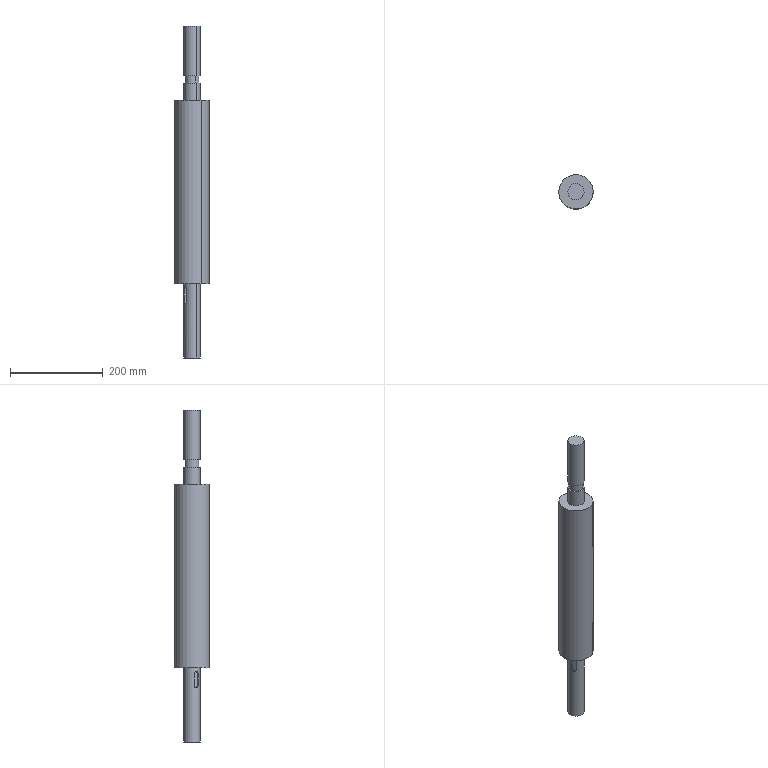Component | SolidWorks | AirShaft-1 | 1 solid | 27 faces | box 74 x 74 x 715 mm | volume 1997791 mm3 | cylinder 14 | plane 9 | cone 4 | commonest cylinder face diameters 35 x6 10.2 x2 30 x2 74 x2 10 x2
build123d program:
from build123d import *

# Parameters (mm, degrees)
SKETCH2_R                              = 17.5
BOSS_EXTRUDE1_DEPTH                    = 160
CUT_EXTRUDE1_REACH                     = 364.802
CUT_EXTRUDE1_END_RADIUS                = 17.5
F_10_2_10_2_DIAMETER_HOLE1_D           = 10.2
F_10_2_10_2_DIAMETER_HOLE1_DEPTH       = 38.75
F_10_2_10_2_DIAMETER_HOLE1_CSINK_D     = 12.05
F_10_2_10_2_DIAMETER_HOLE1_CSINK_ANGLE = 90
F_10_2_10_2_DIAMETER_HOLE1_TIP         = 3.064


with BuildPart() as part:
    # Sketch1 → Revolve1 (revolve)
    with BuildSketch(Plane(origin=(0, 0, 0), x_dir=(-1, 0, 0), z_dir=(0, 0, -1)), mode=Mode.PRIVATE) as revolve1_sk:
        Polygon((-357.5, 17.5), (-357.5, 0), (197.5, 0), (197.5, 37), (-197.5, 37), (-197.5, 17.5), (-234.5, 17.5), (-234.5, 15), (-250.5, 15), (-250.5, 17.5), align=None)
    revolve(revolve1_sk.sketch.rotate(Axis((357.5, 0, 0), (-1, 0, 0)), 270), axis=Axis((357.5, 0, 0), (-1, 0, 0)))

    # Sketch2 → Boss-Extrude1 (add)
    with BuildSketch(Plane.ZY.offset(197.5)):
        Circle(SKETCH2_R)
    extrude(amount=BOSS_EXTRUDE1_DEPTH)

    # Cut-Extrude1: up to this cylinder (the profile starts inside it)
    cut_extrude1_end = Plane(origin=(-223, 0, 0), z_dir=(1, 0, 0)) * Cylinder(CUT_EXTRUDE1_END_RADIUS, 765.604, mode=Mode.PRIVATE)
    # Sketch3 → Cut-Extrude1 (cut, up to the surface)
    with BuildSketch(Plane.XZ.offset(-12.5), mode=Mode.PRIVATE) as cut_extrude1_sk1:
        with BuildLine():
            Line((-235.5, -5), (-210.5, -5))
            ThreePointArc((-210.5, -5), (-205.5, 0), (-210.5, 5))
            Line((-210.5, 5), (-235.5, 5))
            ThreePointArc((-235.5, 5), (-240.5, 0), (-235.5, -5))
        make_face()
    cut_extrude1_tool1 = extrude(cut_extrude1_sk1.sketch, amount=-CUT_EXTRUDE1_REACH, mode=Mode.PRIVATE) & cut_extrude1_end
    add(cut_extrude1_tool1.solids().sort_by_distance((-223, 12.5, 0))[0], mode=Mode.SUBTRACT)

    # 10.2 _10.2_ Diameter Hole1
    with Locations(Plane.ZY.offset(357.5)):
        with Locations((0, 0)):
            CounterSinkHole(F_10_2_10_2_DIAMETER_HOLE1_D / 2, F_10_2_10_2_DIAMETER_HOLE1_CSINK_D / 2, depth=F_10_2_10_2_DIAMETER_HOLE1_DEPTH, counter_sink_angle=F_10_2_10_2_DIAMETER_HOLE1_CSINK_ANGLE)
            with Locations((0, 0, -(F_10_2_10_2_DIAMETER_HOLE1_DEPTH + F_10_2_10_2_DIAMETER_HOLE1_TIP / 2))):  # 118° drill point
                Cone(0, F_10_2_10_2_DIAMETER_HOLE1_D / 2, F_10_2_10_2_DIAMETER_HOLE1_TIP, mode=Mode.SUBTRACT)


solid = part.part

# Placed as in the assembly
solid = solid.moved(Location((-345, -229, 12.5), (90, 31.701, 90)))
STEP:
#1=COLOUR_RGB('',0.7922,0.8196,0.9333);
#2=FILL_AREA_STYLE_COLOUR('',#1);
#3=FILL_AREA_STYLE('',(#2));
#4=SURFACE_STYLE_FILL_AREA(#3);
#5=SURFACE_SIDE_STYLE('',(#4));
#6=SURFACE_STYLE_USAGE(.BOTH.,#5);
#7=PRESENTATION_STYLE_ASSIGNMENT((#6));
#8=CARTESIAN_POINT('',(-13.688,-8.845,-13.546));
#9=VERTEX_POINT('',#8);
#10=CARTESIAN_POINT('',(-13.477,-9.187,-13.546));
#11=VERTEX_POINT('',#10);
#12=CARTESIAN_POINT('',(-13.583,-9.016,-13.546));
#13=DIRECTION('',(0.,0.,-1.));
#14=DIRECTION('',(0.5255,-0.8508,0.));
#15=AXIS2_PLACEMENT_3D('',#12,#13,#14);
#16=CIRCLE('',#15,0.2008);
#17=EDGE_CURVE('',#9,#11,#16,.T.);
#18=ORIENTED_EDGE('',*,*,#17,.F.);
#19=CARTESIAN_POINT('',(-13.707,-8.814,-13.583));
#20=VERTEX_POINT('',#19);
#21=CARTESIAN_POINT('',(-13.707,-8.814,-13.583));
#22=DIRECTION('',(-0.3716,0.6016,-0.7071));
#23=VECTOR('',#22,39.37);
#24=LINE('',#21,#23);
#25=EDGE_CURVE('',#9,#20,#24,.T.);
#26=ORIENTED_EDGE('',*,*,#25,.T.);
#27=CARTESIAN_POINT('',(-13.458,-9.218,-13.583));
#28=VERTEX_POINT('',#27);
#29=CARTESIAN_POINT('',(-13.583,-9.016,-13.583));
#30=DIRECTION('',(0.,0.,-1.));
#31=DIRECTION('',(0.5255,-0.8508,0.));
#32=AXIS2_PLACEMENT_3D('',#29,#30,#31);
#33=CIRCLE('',#32,0.2372);
#34=EDGE_CURVE('',#20,#28,#33,.T.);
#35=ORIENTED_EDGE('',*,*,#34,.T.);
#36=CARTESIAN_POINT('',(-13.458,-9.218,-13.583));
#37=DIRECTION('',(0.3716,-0.6016,-0.7071));
#38=VECTOR('',#37,39.37);
#39=LINE('',#36,#38);
#40=EDGE_CURVE('',#11,#28,#39,.T.);
#41=ORIENTED_EDGE('',*,*,#40,.F.);
#42=EDGE_LOOP('',(#18,#26,#35,#41));
#43=FACE_OUTER_BOUND('',#42,.T.);
#44=CARTESIAN_POINT('',(-13.583,-9.016,-13.583));
#45=DIRECTION('',(0.,0.,-1.));
#46=DIRECTION('',(0.5255,-0.8508,0.));
#47=AXIS2_PLACEMENT_3D('',#44,#45,#46);
#48=CONICAL_SURFACE('',#47,0.2372,0.7854);
#49=ADVANCED_FACE('',(#43),#48,.F.);
#50=CARTESIAN_POINT('',(-13.688,-8.845,-12.057));
#51=VERTEX_POINT('',#50);
#52=CARTESIAN_POINT('',(-13.477,-9.187,-12.057));
#53=VERTEX_POINT('',#52);
#54=CARTESIAN_POINT('',(-13.583,-9.016,-12.057));
#55=DIRECTION('',(0.,0.,-1.));
#56=DIRECTION('',(0.5255,-0.8508,0.));
#57=AXIS2_PLACEMENT_3D('',#54,#55,#56);
#58=CIRCLE('',#57,0.2008);
#59=EDGE_CURVE('',#51,#53,#58,.T.);
#60=ORIENTED_EDGE('',*,*,#59,.F.);
#61=CARTESIAN_POINT('',(-13.688,-8.845,-13.583));
#62=DIRECTION('',(0.,0.,-1.));
#63=VECTOR('',#62,39.37);
#64=LINE('',#61,#63);
#65=EDGE_CURVE('',#51,#9,#64,.T.);
#66=ORIENTED_EDGE('',*,*,#65,.T.);
#67=ORIENTED_EDGE('',*,*,#17,.T.);
#68=CARTESIAN_POINT('',(-13.477,-9.187,-13.583));
#69=DIRECTION('',(0.,0.,-1.));
#70=VECTOR('',#69,39.37);
#71=LINE('',#68,#70);
#72=EDGE_CURVE('',#53,#11,#71,.T.);
#73=ORIENTED_EDGE('',*,*,#72,.F.);
#74=EDGE_LOOP('',(#60,#66,#67,#73));
#75=FACE_OUTER_BOUND('',#74,.T.);
#76=CARTESIAN_POINT('',(-13.583,-9.016,-13.583));
#77=DIRECTION('',(0.,0.,-1.));
#78=DIRECTION('',(0.5255,-0.8508,0.));
#79=AXIS2_PLACEMENT_3D('',#76,#77,#78);
#80=CYLINDRICAL_SURFACE('',#79,0.2008);
#81=ADVANCED_FACE('',(#75),#80,.F.);
#82=CARTESIAN_POINT('',(-13.583,-9.016,-11.936));
#83=VERTEX_POINT('',#82);
#84=CARTESIAN_POINT('',(-13.477,-9.187,-12.057));
#85=DIRECTION('',(0.4504,-0.7293,-0.515));
#86=VECTOR('',#85,39.37);
#87=LINE('',#84,#86);
#88=EDGE_CURVE('',#83,#53,#87,.T.);
#89=ORIENTED_EDGE('',*,*,#88,.F.);
#90=CARTESIAN_POINT('',(-13.688,-8.845,-12.057));
#91=DIRECTION('',(-0.4504,0.7293,-0.515));
#92=VECTOR('',#91,39.37);
#93=LINE('',#90,#92);
#94=EDGE_CURVE('',#83,#51,#93,.T.);
#95=ORIENTED_EDGE('',*,*,#94,.T.);
#96=ORIENTED_EDGE('',*,*,#59,.T.);
#97=EDGE_LOOP('',(#89,#95,#96));
#98=FACE_OUTER_BOUND('',#97,.T.);
#99=CARTESIAN_POINT('',(-13.583,-9.016,-12.057));
#100=DIRECTION('',(0.,0.,-1.));
#101=DIRECTION('',(0.5255,-0.8508,0.));
#102=AXIS2_PLACEMENT_3D('',#99,#100,#101);
#103=CONICAL_SURFACE('',#102,0.2008,1.03);
#104=ADVANCED_FACE('',(#98),#103,.F.);
#105=CARTESIAN_POINT('',(-14.041,-9.53,-7.795));
#106=VERTEX_POINT('',#105);
#107=CARTESIAN_POINT('',(-14.041,-9.53,-8.78));
#108=VERTEX_POINT('',#107);
#109=CARTESIAN_POINT('',(-14.041,-9.53,-13.583));
#110=DIRECTION('',(0.,0.,-1.));
#111=VECTOR('',#110,39.37);
#112=LINE('',#109,#111);
#113=EDGE_CURVE('',#106,#108,#112,.T.);
#114=ORIENTED_EDGE('',*,*,#113,.T.);
#115=CARTESIAN_POINT('',(-14.248,-9.195,-8.78));
#116=VERTEX_POINT('',#115);
#117=CARTESIAN_POINT('',(-14.041,-9.53,-8.78));
#118=CARTESIAN_POINT('',(-14.041,-9.53,-8.793));
#119=CARTESIAN_POINT('',(-14.042,-9.529,-8.805));
#120=CARTESIAN_POINT('',(-14.046,-9.526,-8.831));
#121=CARTESIAN_POINT('',(-14.049,-9.523,-8.843));
#122=CARTESIAN_POINT('',(-14.056,-9.516,-8.867));
#123=CARTESIAN_POINT('',(-14.061,-9.512,-8.878));
#124=CARTESIAN_POINT('',(-14.071,-9.501,-8.9));
#125=CARTESIAN_POINT('',(-14.077,-9.495,-8.91));
#126=CARTESIAN_POINT('',(-14.09,-9.482,-8.928));
#127=CARTESIAN_POINT('',(-14.097,-9.475,-8.936));
#128=CARTESIAN_POINT('',(-14.111,-9.458,-8.95));
#129=CARTESIAN_POINT('',(-14.118,-9.449,-8.956));
#130=CARTESIAN_POINT('',(-14.129,-9.435,-8.964));
#131=CARTESIAN_POINT('',(-14.133,-9.43,-8.966));
#132=CARTESIAN_POINT('',(-14.14,-9.42,-8.97));
#133=CARTESIAN_POINT('',(-14.144,-9.415,-8.971));
#134=CARTESIAN_POINT('',(-14.155,-9.4,-8.975));
#135=CARTESIAN_POINT('',(-14.162,-9.389,-8.976));
#136=CARTESIAN_POINT('',(-14.176,-9.367,-8.976));
#137=CARTESIAN_POINT('',(-14.182,-9.356,-8.975));
#138=CARTESIAN_POINT('',(-14.194,-9.333,-8.97));
#139=CARTESIAN_POINT('',(-14.2,-9.322,-8.966));
#140=CARTESIAN_POINT('',(-14.21,-9.301,-8.956));
#141=CARTESIAN_POINT('',(-14.215,-9.29,-8.95));
#142=CARTESIAN_POINT('',(-14.223,-9.27,-8.936));
#143=CARTESIAN_POINT('',(-14.227,-9.261,-8.928));
#144=CARTESIAN_POINT('',(-14.233,-9.243,-8.91));
#145=CARTESIAN_POINT('',(-14.236,-9.235,-8.9));
#146=CARTESIAN_POINT('',(-14.24,-9.221,-8.879));
#147=CARTESIAN_POINT('',(-14.242,-9.215,-8.867));
#148=CARTESIAN_POINT('',(-14.245,-9.205,-8.843));
#149=CARTESIAN_POINT('',(-14.246,-9.202,-8.831));
#150=CARTESIAN_POINT('',(-14.248,-9.197,-8.806));
#151=CARTESIAN_POINT('',(-14.248,-9.195,-8.793));
#152=CARTESIAN_POINT('',(-14.248,-9.195,-8.78));
#153=B_SPLINE_CURVE_WITH_KNOTS('',3,(#117,#118,#119,#120,#121,#122,#123,#124,#125,#126,#127,#128,#129,#130,#131,#132,#133,#134,#135,#136,#137,#138,#139,#140,#141,#142,#143,#144,#145,#146,#147,#148,#149,#150,#151,#152),.UNSPECIFIED.,.F.,.F.,(4,2,2,2,2,2,2,2,2,2,2,2,2,2,2,2,2,4),(0.,0.0009818,0.001964,0.002945,0.003927,0.004909,0.005891,0.006382,0.006873,0.007855,0.008836,0.009818,0.0108,0.01178,0.01276,0.01375,0.01473,0.01571),.UNSPECIFIED.);
#154=EDGE_CURVE('',#108,#116,#153,.T.);
#155=ORIENTED_EDGE('',*,*,#154,.T.);
#156=CARTESIAN_POINT('',(-14.248,-9.195,-7.795));
#157=VERTEX_POINT('',#156);
#158=CARTESIAN_POINT('',(-14.248,-9.195,-13.583));
#159=DIRECTION('',(-0.,-0.,1.));
#160=VECTOR('',#159,39.37);
#161=LINE('',#158,#160);
#162=EDGE_CURVE('',#116,#157,#161,.T.);
#163=ORIENTED_EDGE('',*,*,#162,.T.);
#164=CARTESIAN_POINT('',(-14.248,-9.195,-7.795));
#165=CARTESIAN_POINT('',(-14.248,-9.195,-7.782));
#166=CARTESIAN_POINT('',(-14.248,-9.197,-7.769));
#167=CARTESIAN_POINT('',(-14.246,-9.202,-7.744));
#168=CARTESIAN_POINT('',(-14.245,-9.205,-7.732));
#169=CARTESIAN_POINT('',(-14.242,-9.215,-7.708));
#170=CARTESIAN_POINT('',(-14.24,-9.221,-7.697));
#171=CARTESIAN_POINT('',(-14.236,-9.235,-7.675));
#172=CARTESIAN_POINT('',(-14.233,-9.243,-7.665));
#173=CARTESIAN_POINT('',(-14.227,-9.261,-7.647));
#174=CARTESIAN_POINT('',(-14.223,-9.27,-7.639));
#175=CARTESIAN_POINT('',(-14.215,-9.29,-7.625));
#176=CARTESIAN_POINT('',(-14.21,-9.3,-7.618));
#177=CARTESIAN_POINT('',(-14.203,-9.317,-7.611));
#178=CARTESIAN_POINT('',(-14.2,-9.322,-7.609));
#179=CARTESIAN_POINT('',(-14.194,-9.333,-7.605));
#180=CARTESIAN_POINT('',(-14.191,-9.339,-7.604));
#181=CARTESIAN_POINT('',(-14.182,-9.356,-7.6));
#182=CARTESIAN_POINT('',(-14.176,-9.367,-7.598));
#183=CARTESIAN_POINT('',(-14.162,-9.389,-7.598));
#184=CARTESIAN_POINT('',(-14.155,-9.4,-7.6));
#185=CARTESIAN_POINT('',(-14.14,-9.42,-7.605));
#186=CARTESIAN_POINT('',(-14.133,-9.43,-7.608));
#187=CARTESIAN_POINT('',(-14.118,-9.449,-7.618));
#188=CARTESIAN_POINT('',(-14.111,-9.458,-7.625));
#189=CARTESIAN_POINT('',(-14.097,-9.474,-7.639));
#190=CARTESIAN_POINT('',(-14.09,-9.482,-7.647));
#191=CARTESIAN_POINT('',(-14.077,-9.495,-7.665));
#192=CARTESIAN_POINT('',(-14.071,-9.501,-7.675));
#193=CARTESIAN_POINT('',(-14.061,-9.512,-7.696));
#194=CARTESIAN_POINT('',(-14.056,-9.516,-7.708));
#195=CARTESIAN_POINT('',(-14.049,-9.523,-7.731));
#196=CARTESIAN_POINT('',(-14.046,-9.526,-7.744));
#197=CARTESIAN_POINT('',(-14.042,-9.529,-7.769));
#198=CARTESIAN_POINT('',(-14.041,-9.53,-7.782));
#199=CARTESIAN_POINT('',(-14.041,-9.53,-7.795));
#200=B_SPLINE_CURVE_WITH_KNOTS('',3,(#164,#165,#166,#167,#168,#169,#170,#171,#172,#173,#174,#175,#176,#177,#178,#179,#180,#181,#182,#183,#184,#185,#186,#187,#188,#189,#190,#191,#192,#193,#194,#195,#196,#197,#198,#199),.UNSPECIFIED.,.F.,.F.,(4,2,2,2,2,2,2,2,2,2,2,2,2,2,2,2,2,4),(0.,0.0009818,0.001964,0.002945,0.003927,0.004909,0.005891,0.006382,0.006873,0.007855,0.008836,0.009818,0.0108,0.01178,0.01276,0.01375,0.01473,0.01571),.UNSPECIFIED.);
#201=EDGE_CURVE('',#157,#106,#200,.T.);
#202=ORIENTED_EDGE('',*,*,#201,.T.);
#203=EDGE_LOOP('',(#114,#155,#163,#202));
#204=FACE_BOUND('',#203,.T.);
#205=CARTESIAN_POINT('',(-13.221,-9.602,-13.583));
#206=VERTEX_POINT('',#205);
#207=CARTESIAN_POINT('',(-13.945,-8.43,-13.583));
#208=VERTEX_POINT('',#207);
#209=CARTESIAN_POINT('',(-13.583,-9.016,-13.583));
#210=DIRECTION('',(0.,0.,-1.));
#211=DIRECTION('',(0.5255,-0.8508,0.));
#212=AXIS2_PLACEMENT_3D('',#209,#210,#211);
#213=CIRCLE('',#212,0.689);
#214=EDGE_CURVE('',#206,#208,#213,.T.);
#215=ORIENTED_EDGE('',*,*,#214,.F.);
#216=CARTESIAN_POINT('',(-13.221,-9.602,-7.283));
#217=VERTEX_POINT('',#216);
#218=CARTESIAN_POINT('',(-13.221,-9.602,-13.583));
#219=DIRECTION('',(-0.,-0.,1.));
#220=VECTOR('',#219,39.37);
#221=LINE('',#218,#220);
#222=EDGE_CURVE('',#206,#217,#221,.T.);
#223=ORIENTED_EDGE('',*,*,#222,.T.);
#224=CARTESIAN_POINT('',(-13.945,-8.43,-7.283));
#225=VERTEX_POINT('',#224);
#226=CARTESIAN_POINT('',(-13.583,-9.016,-7.283));
#227=DIRECTION('',(0.,0.,-1.));
#228=DIRECTION('',(0.5255,-0.8508,0.));
#229=AXIS2_PLACEMENT_3D('',#226,#227,#228);
#230=CIRCLE('',#229,0.689);
#231=EDGE_CURVE('',#217,#225,#230,.T.);
#232=ORIENTED_EDGE('',*,*,#231,.T.);
#233=CARTESIAN_POINT('',(-13.945,-8.43,-13.583));
#234=DIRECTION('',(-0.,-0.,1.));
#235=VECTOR('',#234,39.37);
#236=LINE('',#233,#235);
#237=EDGE_CURVE('',#208,#225,#236,.T.);
#238=ORIENTED_EDGE('',*,*,#237,.F.);
#239=EDGE_LOOP('',(#215,#223,#232,#238));
#240=FACE_OUTER_BOUND('',#239,.T.);
#241=CARTESIAN_POINT('',(-13.583,-9.016,-13.583));
#242=DIRECTION('',(-0.,-0.,1.));
#243=DIRECTION('',(-0.5255,0.8508,0.));
#244=AXIS2_PLACEMENT_3D('',#241,#242,#243);
#245=CYLINDRICAL_SURFACE('',#244,0.689);
#246=ADVANCED_FACE('',(#204,#240),#245,.T.);
#247=CARTESIAN_POINT('',(-13.272,-9.518,10.354));
#248=VERTEX_POINT('',#247);
#249=CARTESIAN_POINT('',(-13.893,-8.513,10.354));
#250=VERTEX_POINT('',#249);
#251=CARTESIAN_POINT('',(-13.583,-9.016,10.354));
#252=DIRECTION('',(0.,0.,-1.));
#253=DIRECTION('',(0.5255,-0.8508,0.));
#254=AXIS2_PLACEMENT_3D('',#251,#252,#253);
#255=CIRCLE('',#254,0.5906);
#256=EDGE_CURVE('',#248,#250,#255,.T.);
#257=ORIENTED_EDGE('',*,*,#256,.T.);
#258=CARTESIAN_POINT('',(-13.893,-8.513,9.724));
#259=VERTEX_POINT('',#258);
#260=CARTESIAN_POINT('',(-13.893,-8.513,14.567));
#261=DIRECTION('',(0.,0.,-1.));
#262=VECTOR('',#261,39.37);
#263=LINE('',#260,#262);
#264=EDGE_CURVE('',#250,#259,#263,.T.);
#265=ORIENTED_EDGE('',*,*,#264,.T.);
#266=CARTESIAN_POINT('',(-13.272,-9.518,9.724));
#267=VERTEX_POINT('',#266);
#268=CARTESIAN_POINT('',(-13.583,-9.016,9.724));
#269=DIRECTION('',(0.,0.,-1.));
#270=DIRECTION('',(0.5255,-0.8508,0.));
#271=AXIS2_PLACEMENT_3D('',#268,#269,#270);
#272=CIRCLE('',#271,0.5906);
#273=EDGE_CURVE('',#267,#259,#272,.T.);
#274=ORIENTED_EDGE('',*,*,#273,.F.);
#275=CARTESIAN_POINT('',(-13.272,-9.518,14.567));
#276=DIRECTION('',(0.,0.,-1.));
#277=VECTOR('',#276,39.37);
#278=LINE('',#275,#277);
#279=EDGE_CURVE('',#248,#267,#278,.T.);
#280=ORIENTED_EDGE('',*,*,#279,.F.);
#281=EDGE_LOOP('',(#257,#265,#274,#280));
#282=FACE_OUTER_BOUND('',#281,.T.);
#283=CARTESIAN_POINT('',(-13.583,-9.016,14.567));
#284=DIRECTION('',(0.,0.,-1.));
#285=DIRECTION('',(0.5255,-0.8508,0.));
#286=AXIS2_PLACEMENT_3D('',#283,#284,#285);
#287=CYLINDRICAL_SURFACE('',#286,0.5906);
#288=ADVANCED_FACE('',(#282),#287,.T.);
#289=CARTESIAN_POINT('',(-13.221,-9.602,9.724));
#290=VERTEX_POINT('',#289);
#291=CARTESIAN_POINT('',(-13.945,-8.43,9.724));
#292=VERTEX_POINT('',#291);
#293=CARTESIAN_POINT('',(-13.583,-9.016,9.724));
#294=DIRECTION('',(0.,0.,-1.));
#295=DIRECTION('',(0.5255,-0.8508,0.));
#296=AXIS2_PLACEMENT_3D('',#293,#294,#295);
#297=CIRCLE('',#296,0.689);
#298=EDGE_CURVE('',#290,#292,#297,.T.);
#299=ORIENTED_EDGE('',*,*,#298,.T.);
#300=CARTESIAN_POINT('',(-13.945,-8.43,8.268));
#301=VERTEX_POINT('',#300);
#302=CARTESIAN_POINT('',(-13.945,-8.43,14.567));
#303=DIRECTION('',(0.,0.,-1.));
#304=VECTOR('',#303,39.37);
#305=LINE('',#302,#304);
#306=EDGE_CURVE('',#292,#301,#305,.T.);
#307=ORIENTED_EDGE('',*,*,#306,.T.);
#308=CARTESIAN_POINT('',(-13.221,-9.602,8.268));
#309=VERTEX_POINT('',#308);
#310=CARTESIAN_POINT('',(-13.583,-9.016,8.268));
#311=DIRECTION('',(0.,0.,-1.));
#312=DIRECTION('',(0.5255,-0.8508,0.));
#313=AXIS2_PLACEMENT_3D('',#310,#311,#312);
#314=CIRCLE('',#313,0.689);
#315=EDGE_CURVE('',#309,#301,#314,.T.);
#316=ORIENTED_EDGE('',*,*,#315,.F.);
#317=CARTESIAN_POINT('',(-13.221,-9.602,14.567));
#318=DIRECTION('',(0.,0.,-1.));
#319=VECTOR('',#318,39.37);
#320=LINE('',#317,#319);
#321=EDGE_CURVE('',#290,#309,#320,.T.);
#322=ORIENTED_EDGE('',*,*,#321,.F.);
#323=EDGE_LOOP('',(#299,#307,#316,#322));
#324=FACE_OUTER_BOUND('',#323,.T.);
#325=CARTESIAN_POINT('',(-13.583,-9.016,14.567));
#326=DIRECTION('',(0.,0.,-1.));
#327=DIRECTION('',(0.5255,-0.8508,0.));
#328=AXIS2_PLACEMENT_3D('',#325,#326,#327);
#329=CYLINDRICAL_SURFACE('',#328,0.689);
#330=ADVANCED_FACE('',(#324),#329,.T.);
#331=CARTESIAN_POINT('',(-12.817,-10.255,8.268));
#332=VERTEX_POINT('',#331);
#333=CARTESIAN_POINT('',(-14.348,-7.776,8.268));
#334=VERTEX_POINT('',#333);
#335=CARTESIAN_POINT('',(-13.583,-9.016,8.268));
#336=DIRECTION('',(0.,0.,-1.));
#337=DIRECTION('',(0.5255,-0.8508,0.));
#338=AXIS2_PLACEMENT_3D('',#335,#336,#337);
#339=CIRCLE('',#338,1.457);
#340=EDGE_CURVE('',#332,#334,#339,.T.);
#341=ORIENTED_EDGE('',*,*,#340,.T.);
#342=CARTESIAN_POINT('',(-14.348,-7.776,-7.283));
#343=VERTEX_POINT('',#342);
#344=CARTESIAN_POINT('',(-14.348,-7.776,14.567));
#345=DIRECTION('',(0.,0.,-1.));
#346=VECTOR('',#345,39.37);
#347=LINE('',#344,#346);
#348=EDGE_CURVE('',#334,#343,#347,.T.);
#349=ORIENTED_EDGE('',*,*,#348,.T.);
#350=CARTESIAN_POINT('',(-12.817,-10.255,-7.283));
#351=VERTEX_POINT('',#350);
#352=CARTESIAN_POINT('',(-13.583,-9.016,-7.283));
#353=DIRECTION('',(0.,0.,-1.));
#354=DIRECTION('',(0.5255,-0.8508,0.));
#355=AXIS2_PLACEMENT_3D('',#352,#353,#354);
#356=CIRCLE('',#355,1.457);
#357=EDGE_CURVE('',#351,#343,#356,.T.);
#358=ORIENTED_EDGE('',*,*,#357,.F.);
#359=CARTESIAN_POINT('',(-12.817,-10.255,14.567));
#360=DIRECTION('',(0.,0.,-1.));
#361=VECTOR('',#360,39.37);
#362=LINE('',#359,#361);
#363=EDGE_CURVE('',#332,#351,#362,.T.);
#364=ORIENTED_EDGE('',*,*,#363,.F.);
#365=EDGE_LOOP('',(#341,#349,#358,#364));
#366=FACE_OUTER_BOUND('',#365,.T.);
#367=CARTESIAN_POINT('',(-13.583,-9.016,14.567));
#368=DIRECTION('',(0.,0.,-1.));
#369=DIRECTION('',(0.5255,-0.8508,0.));
#370=AXIS2_PLACEMENT_3D('',#367,#368,#369);
#371=CYLINDRICAL_SURFACE('',#370,1.457);
#372=ADVANCED_FACE('',(#366),#371,.T.);
#373=CARTESIAN_POINT('',(-13.221,-9.602,14.567));
#374=VERTEX_POINT('',#373);
#375=CARTESIAN_POINT('',(-13.945,-8.43,14.567));
#376=VERTEX_POINT('',#375);
#377=CARTESIAN_POINT('',(-13.583,-9.016,14.567));
#378=DIRECTION('',(0.,0.,-1.));
#379=DIRECTION('',(0.5255,-0.8508,0.));
#380=AXIS2_PLACEMENT_3D('',#377,#378,#379);
#381=CIRCLE('',#380,0.689);
#382=EDGE_CURVE('',#374,#376,#381,.T.);
#383=ORIENTED_EDGE('',*,*,#382,.T.);
#384=CARTESIAN_POINT('',(-13.945,-8.43,10.354));
#385=VERTEX_POINT('',#384);
#386=CARTESIAN_POINT('',(-13.945,-8.43,14.567));
#387=DIRECTION('',(0.,0.,-1.));
#388=VECTOR('',#387,39.37);
#389=LINE('',#386,#388);
#390=EDGE_CURVE('',#376,#385,#389,.T.);
#391=ORIENTED_EDGE('',*,*,#390,.T.);
#392=CARTESIAN_POINT('',(-13.221,-9.602,10.354));
#393=VERTEX_POINT('',#392);
#394=CARTESIAN_POINT('',(-13.583,-9.016,10.354));
#395=DIRECTION('',(0.,0.,-1.));
#396=DIRECTION('',(0.5255,-0.8508,0.));
#397=AXIS2_PLACEMENT_3D('',#394,#395,#396);
#398=CIRCLE('',#397,0.689);
#399=EDGE_CURVE('',#393,#385,#398,.T.);
#400=ORIENTED_EDGE('',*,*,#399,.F.);
#401=CARTESIAN_POINT('',(-13.221,-9.602,14.567));
#402=DIRECTION('',(0.,0.,-1.));
#403=VECTOR('',#402,39.37);
#404=LINE('',#401,#403);
#405=EDGE_CURVE('',#374,#393,#404,.T.);
#406=ORIENTED_EDGE('',*,*,#405,.F.);
#407=EDGE_LOOP('',(#383,#391,#400,#406));
#408=FACE_OUTER_BOUND('',#407,.T.);
#409=CARTESIAN_POINT('',(-13.583,-9.016,14.567));
#410=DIRECTION('',(0.,0.,-1.));
#411=DIRECTION('',(0.5255,-0.8508,0.));
#412=AXIS2_PLACEMENT_3D('',#409,#410,#411);
#413=CYLINDRICAL_SURFACE('',#412,0.689);
#414=ADVANCED_FACE('',(#408),#413,.T.);
#415=ORIENTED_EDGE('',*,*,#390,.F.);
#416=CARTESIAN_POINT('',(-13.583,-9.016,14.567));
#417=DIRECTION('',(0.,0.,-1.));
#418=DIRECTION('',(0.5255,-0.8508,0.));
#419=AXIS2_PLACEMENT_3D('',#416,#417,#418);
#420=CIRCLE('',#419,0.689);
#421=EDGE_CURVE('',#376,#374,#420,.T.);
#422=ORIENTED_EDGE('',*,*,#421,.T.);
#423=ORIENTED_EDGE('',*,*,#405,.T.);
#424=CARTESIAN_POINT('',(-13.583,-9.016,10.354));
#425=DIRECTION('',(0.,0.,-1.));
#426=DIRECTION('',(0.5255,-0.8508,0.));
#427=AXIS2_PLACEMENT_3D('',#424,#425,#426);
#428=CIRCLE('',#427,0.689);
#429=EDGE_CURVE('',#385,#393,#428,.T.);
#430=ORIENTED_EDGE('',*,*,#429,.F.);
#431=EDGE_LOOP('',(#415,#422,#423,#430));
#432=FACE_OUTER_BOUND('',#431,.T.);
#433=CARTESIAN_POINT('',(-13.583,-9.016,14.567));
#434=DIRECTION('',(0.,0.,-1.));
#435=DIRECTION('',(0.5255,-0.8508,0.));
#436=AXIS2_PLACEMENT_3D('',#433,#434,#435);
#437=CYLINDRICAL_SURFACE('',#436,0.689);
#438=ADVANCED_FACE('',(#432),#437,.T.);
#439=ORIENTED_EDGE('',*,*,#382,.F.);
#440=ORIENTED_EDGE('',*,*,#421,.F.);
#441=EDGE_LOOP('',(#439,#440));
#442=FACE_OUTER_BOUND('',#441,.T.);
#443=CARTESIAN_POINT('',(-14.169,-9.378,14.567));
#444=DIRECTION('',(-0.,-0.,1.));
#445=DIRECTION('',(-0.5255,0.8508,0.));
#446=AXIS2_PLACEMENT_3D('',#443,#444,#445);
#447=PLANE('',#446);
#448=ADVANCED_FACE('',(#442),#447,.T.);
#449=CARTESIAN_POINT('',(-13.583,-9.016,-7.283));
#450=DIRECTION('',(0.,0.,-1.));
#451=DIRECTION('',(0.5255,-0.8508,0.));
#452=AXIS2_PLACEMENT_3D('',#449,#450,#451);
#453=CIRCLE('',#452,0.689);
#454=EDGE_CURVE('',#225,#217,#453,.T.);
#455=ORIENTED_EDGE('',*,*,#454,.F.);
#456=ORIENTED_EDGE('',*,*,#231,.F.);
#457=EDGE_LOOP('',(#455,#456));
#458=FACE_BOUND('',#457,.T.);
#459=ORIENTED_EDGE('',*,*,#357,.T.);
#460=CARTESIAN_POINT('',(-13.583,-9.016,-7.283));
#461=DIRECTION('',(0.,0.,-1.));
#462=DIRECTION('',(0.5255,-0.8508,0.));
#463=AXIS2_PLACEMENT_3D('',#460,#461,#462);
#464=CIRCLE('',#463,1.457);
#465=EDGE_CURVE('',#343,#351,#464,.T.);
#466=ORIENTED_EDGE('',*,*,#465,.T.);
#467=EDGE_LOOP('',(#459,#466));
#468=FACE_OUTER_BOUND('',#467,.T.);
#469=CARTESIAN_POINT('',(-13.583,-9.016,-7.283));
#470=DIRECTION('',(0.,0.,-1.));
#471=DIRECTION('',(0.5255,-0.8508,0.));
#472=AXIS2_PLACEMENT_3D('',#469,#470,#471);
#473=PLANE('',#472);
#474=ADVANCED_FACE('',(#458,#468),#473,.T.);
#475=ORIENTED_EDGE('',*,*,#348,.F.);
#476=CARTESIAN_POINT('',(-13.583,-9.016,8.268));
#477=DIRECTION('',(0.,0.,-1.));
#478=DIRECTION('',(0.5255,-0.8508,0.));
#479=AXIS2_PLACEMENT_3D('',#476,#477,#478);
#480=CIRCLE('',#479,1.457);
#481=EDGE_CURVE('',#334,#332,#480,.T.);
#482=ORIENTED_EDGE('',*,*,#481,.T.);
#483=ORIENTED_EDGE('',*,*,#363,.T.);
#484=ORIENTED_EDGE('',*,*,#465,.F.);
#485=EDGE_LOOP('',(#475,#482,#483,#484));
#486=FACE_OUTER_BOUND('',#485,.T.);
#487=CARTESIAN_POINT('',(-13.583,-9.016,14.567));
#488=DIRECTION('',(0.,0.,-1.));
#489=DIRECTION('',(0.5255,-0.8508,0.));
#490=AXIS2_PLACEMENT_3D('',#487,#488,#489);
#491=CYLINDRICAL_SURFACE('',#490,1.457);
#492=ADVANCED_FACE('',(#486),#491,.T.);
#493=ORIENTED_EDGE('',*,*,#315,.T.);
#494=CARTESIAN_POINT('',(-13.583,-9.016,8.268));
#495=DIRECTION('',(0.,0.,-1.));
#496=DIRECTION('',(0.5255,-0.8508,0.));
#497=AXIS2_PLACEMENT_3D('',#494,#495,#496);
#498=CIRCLE('',#497,0.689);
#499=EDGE_CURVE('',#301,#309,#498,.T.);
#500=ORIENTED_EDGE('',*,*,#499,.T.);
#501=EDGE_LOOP('',(#493,#500));
#502=FACE_BOUND('',#501,.T.);
#503=ORIENTED_EDGE('',*,*,#340,.F.);
#504=ORIENTED_EDGE('',*,*,#481,.F.);
#505=EDGE_LOOP('',(#503,#504));
#506=FACE_OUTER_BOUND('',#505,.T.);
#507=CARTESIAN_POINT('',(-14.822,-9.781,8.268));
#508=DIRECTION('',(-0.,-0.,1.));
#509=DIRECTION('',(-0.5255,0.8508,0.));
#510=AXIS2_PLACEMENT_3D('',#507,#508,#509);
#511=PLANE('',#510);
#512=ADVANCED_FACE('',(#502,#506),#511,.T.);
#513=ORIENTED_EDGE('',*,*,#306,.F.);
#514=CARTESIAN_POINT('',(-13.583,-9.016,9.724));
#515=DIRECTION('',(0.,0.,-1.));
#516=DIRECTION('',(0.5255,-0.8508,0.));
#517=AXIS2_PLACEMENT_3D('',#514,#515,#516);
#518=CIRCLE('',#517,0.689);
#519=EDGE_CURVE('',#292,#290,#518,.T.);
#520=ORIENTED_EDGE('',*,*,#519,.T.);
#521=ORIENTED_EDGE('',*,*,#321,.T.);
#522=ORIENTED_EDGE('',*,*,#499,.F.);
#523=EDGE_LOOP('',(#513,#520,#521,#522));
#524=FACE_OUTER_BOUND('',#523,.T.);
#525=CARTESIAN_POINT('',(-13.583,-9.016,14.567));
#526=DIRECTION('',(0.,0.,-1.));
#527=DIRECTION('',(0.5255,-0.8508,0.));
#528=AXIS2_PLACEMENT_3D('',#525,#526,#527);
#529=CYLINDRICAL_SURFACE('',#528,0.689);
#530=ADVANCED_FACE('',(#524),#529,.T.);
#531=ORIENTED_EDGE('',*,*,#273,.T.);
#532=CARTESIAN_POINT('',(-13.583,-9.016,9.724));
#533=DIRECTION('',(0.,0.,-1.));
#534=DIRECTION('',(0.5255,-0.8508,0.));
#535=AXIS2_PLACEMENT_3D('',#532,#533,#534);
#536=CIRCLE('',#535,0.5906);
#537=EDGE_CURVE('',#259,#267,#536,.T.);
#538=ORIENTED_EDGE('',*,*,#537,.T.);
#539=EDGE_LOOP('',(#531,#538));
#540=FACE_BOUND('',#539,.T.);
#541=ORIENTED_EDGE('',*,*,#298,.F.);
#542=ORIENTED_EDGE('',*,*,#519,.F.);
#543=EDGE_LOOP('',(#541,#542));
#544=FACE_OUTER_BOUND('',#543,.T.);
#545=CARTESIAN_POINT('',(-14.169,-9.378,9.724));
#546=DIRECTION('',(-0.,-0.,1.));
#547=DIRECTION('',(-0.5255,0.8508,0.));
#548=AXIS2_PLACEMENT_3D('',#545,#546,#547);
#549=PLANE('',#548);
#550=ADVANCED_FACE('',(#540,#544),#549,.T.);
#551=ORIENTED_EDGE('',*,*,#264,.F.);
#552=CARTESIAN_POINT('',(-13.583,-9.016,10.354));
#553=DIRECTION('',(0.,0.,-1.));
#554=DIRECTION('',(0.5255,-0.8508,0.));
#555=AXIS2_PLACEMENT_3D('',#552,#553,#554);
#556=CIRCLE('',#555,0.5906);
#557=EDGE_CURVE('',#250,#248,#556,.T.);
#558=ORIENTED_EDGE('',*,*,#557,.T.);
#559=ORIENTED_EDGE('',*,*,#279,.T.);
#560=ORIENTED_EDGE('',*,*,#537,.F.);
#561=EDGE_LOOP('',(#551,#558,#559,#560));
#562=FACE_OUTER_BOUND('',#561,.T.);
#563=CARTESIAN_POINT('',(-13.583,-9.016,14.567));
#564=DIRECTION('',(0.,0.,-1.));
#565=DIRECTION('',(0.5255,-0.8508,0.));
#566=AXIS2_PLACEMENT_3D('',#563,#564,#565);
#567=CYLINDRICAL_SURFACE('',#566,0.5906);
#568=ADVANCED_FACE('',(#562),#567,.T.);
#569=ORIENTED_EDGE('',*,*,#399,.T.);
#570=ORIENTED_EDGE('',*,*,#429,.T.);
#571=EDGE_LOOP('',(#569,#570));
#572=FACE_OUTER_BOUND('',#571,.T.);
#573=ORIENTED_EDGE('',*,*,#256,.F.);
#574=ORIENTED_EDGE('',*,*,#557,.F.);
#575=EDGE_LOOP('',(#573,#574));
#576=FACE_BOUND('',#575,.T.);
#577=CARTESIAN_POINT('',(-14.085,-9.326,10.354));
#578=DIRECTION('',(0.,0.,-1.));
#579=DIRECTION('',(0.5255,-0.8508,0.));
#580=AXIS2_PLACEMENT_3D('',#577,#578,#579);
#581=PLANE('',#580);
#582=ADVANCED_FACE('',(#572,#576),#581,.T.);
#583=ORIENTED_EDGE('',*,*,#222,.F.);
#584=CARTESIAN_POINT('',(-13.583,-9.016,-13.583));
#585=DIRECTION('',(0.,0.,-1.));
#586=DIRECTION('',(0.5255,-0.8508,0.));
#587=AXIS2_PLACEMENT_3D('',#584,#585,#586);
#588=CIRCLE('',#587,0.689);
#589=EDGE_CURVE('',#208,#206,#588,.T.);
#590=ORIENTED_EDGE('',*,*,#589,.F.);
#591=ORIENTED_EDGE('',*,*,#237,.T.);
#592=ORIENTED_EDGE('',*,*,#454,.T.);
#593=EDGE_LOOP('',(#583,#590,#591,#592));
#594=FACE_OUTER_BOUND('',#593,.T.);
#595=CARTESIAN_POINT('',(-13.583,-9.016,-13.583));
#596=DIRECTION('',(-0.,-0.,1.));
#597=DIRECTION('',(-0.5255,0.8508,0.));
#598=AXIS2_PLACEMENT_3D('',#595,#596,#597);
#599=CYLINDRICAL_SURFACE('',#598,0.689);
#600=ADVANCED_FACE('',(#594),#599,.T.);
#601=CARTESIAN_POINT('',(-13.583,-9.016,-13.583));
#602=DIRECTION('',(0.,0.,-1.));
#603=DIRECTION('',(0.5255,-0.8508,0.));
#604=AXIS2_PLACEMENT_3D('',#601,#602,#603);
#605=CIRCLE('',#604,0.2372);
#606=EDGE_CURVE('',#28,#20,#605,.T.);
#607=ORIENTED_EDGE('',*,*,#606,.F.);
#608=ORIENTED_EDGE('',*,*,#34,.F.);
#609=EDGE_LOOP('',(#607,#608));
#610=FACE_BOUND('',#609,.T.);
#611=ORIENTED_EDGE('',*,*,#589,.T.);
#612=ORIENTED_EDGE('',*,*,#214,.T.);
#613=EDGE_LOOP('',(#611,#612));
#614=FACE_OUTER_BOUND('',#613,.T.);
#615=CARTESIAN_POINT('',(-13.583,-9.016,-13.583));
#616=DIRECTION('',(0.,0.,-1.));
#617=DIRECTION('',(0.5255,-0.8508,0.));
#618=AXIS2_PLACEMENT_3D('',#615,#616,#617);
#619=PLANE('',#618);
#620=ADVANCED_FACE('',(#610,#614),#619,.T.);
#621=ORIENTED_EDGE('',*,*,#154,.F.);
#622=CARTESIAN_POINT('',(-13.898,-9.442,-8.78));
#623=VERTEX_POINT('',#622);
#624=CARTESIAN_POINT('',(-14.719,-9.949,-8.78));
#625=DIRECTION('',(0.8508,0.5255,0.));
#626=VECTOR('',#625,39.37);
#627=LINE('',#624,#626);
#628=EDGE_CURVE('',#108,#623,#627,.T.);
#629=ORIENTED_EDGE('',*,*,#628,.T.);
#630=CARTESIAN_POINT('',(-14.105,-9.107,-8.78));
#631=VERTEX_POINT('',#630);
#632=CARTESIAN_POINT('',(-14.001,-9.274,-8.78));
#633=DIRECTION('',(0.8508,0.5255,0.));
#634=DIRECTION('',(-0.5255,0.8508,0.));
#635=AXIS2_PLACEMENT_3D('',#632,#633,#634);
#636=CIRCLE('',#635,0.1969);
#637=EDGE_CURVE('',#623,#631,#636,.T.);
#638=ORIENTED_EDGE('',*,*,#637,.T.);
#639=CARTESIAN_POINT('',(-14.926,-9.614,-8.78));
#640=DIRECTION('',(0.8508,0.5255,0.));
#641=VECTOR('',#640,39.37);
#642=LINE('',#639,#641);
#643=EDGE_CURVE('',#116,#631,#642,.T.);
#644=ORIENTED_EDGE('',*,*,#643,.F.);
#645=EDGE_LOOP('',(#621,#629,#638,#644));
#646=FACE_OUTER_BOUND('',#645,.T.);
#647=CARTESIAN_POINT('',(-14.822,-9.781,-8.78));
#648=DIRECTION('',(0.8508,0.5255,0.));
#649=DIRECTION('',(-0.5255,0.8508,0.));
#650=AXIS2_PLACEMENT_3D('',#647,#648,#649);
#651=CYLINDRICAL_SURFACE('',#650,0.1969);
#652=ADVANCED_FACE('',(#646),#651,.F.);
#653=ORIENTED_EDGE('',*,*,#113,.F.);
#654=CARTESIAN_POINT('',(-13.898,-9.442,-7.795));
#655=VERTEX_POINT('',#654);
#656=CARTESIAN_POINT('',(-14.719,-9.949,-7.795));
#657=DIRECTION('',(0.8508,0.5255,0.));
#658=VECTOR('',#657,39.37);
#659=LINE('',#656,#658);
#660=EDGE_CURVE('',#106,#655,#659,.T.);
#661=ORIENTED_EDGE('',*,*,#660,.T.);
#662=CARTESIAN_POINT('',(-13.898,-9.442,-7.795));
#663=DIRECTION('',(0.,-0.,-1.));
#664=VECTOR('',#663,39.37);
#665=LINE('',#662,#664);
#666=EDGE_CURVE('',#655,#623,#665,.T.);
#667=ORIENTED_EDGE('',*,*,#666,.T.);
#668=ORIENTED_EDGE('',*,*,#628,.F.);
#669=EDGE_LOOP('',(#653,#661,#667,#668));
#670=FACE_OUTER_BOUND('',#669,.T.);
#671=CARTESIAN_POINT('',(-14.719,-9.949,-7.795));
#672=DIRECTION('',(0.5255,-0.8508,0.));
#673=DIRECTION('',(-0.,0.,1.));
#674=AXIS2_PLACEMENT_3D('',#671,#672,#673);
#675=PLANE('',#674);
#676=ADVANCED_FACE('',(#670),#675,.F.);
#677=ORIENTED_EDGE('',*,*,#201,.F.);
#678=CARTESIAN_POINT('',(-14.105,-9.107,-7.795));
#679=VERTEX_POINT('',#678);
#680=CARTESIAN_POINT('',(-14.926,-9.614,-7.795));
#681=DIRECTION('',(0.8508,0.5255,0.));
#682=VECTOR('',#681,39.37);
#683=LINE('',#680,#682);
#684=EDGE_CURVE('',#157,#679,#683,.T.);
#685=ORIENTED_EDGE('',*,*,#684,.T.);
#686=CARTESIAN_POINT('',(-14.001,-9.274,-7.795));
#687=DIRECTION('',(0.8508,0.5255,0.));
#688=DIRECTION('',(-0.5255,0.8508,0.));
#689=AXIS2_PLACEMENT_3D('',#686,#687,#688);
#690=CIRCLE('',#689,0.1969);
#691=EDGE_CURVE('',#679,#655,#690,.T.);
#692=ORIENTED_EDGE('',*,*,#691,.T.);
#693=ORIENTED_EDGE('',*,*,#660,.F.);
#694=EDGE_LOOP('',(#677,#685,#692,#693));
#695=FACE_OUTER_BOUND('',#694,.T.);
#696=CARTESIAN_POINT('',(-14.822,-9.781,-7.795));
#697=DIRECTION('',(0.8508,0.5255,0.));
#698=DIRECTION('',(-0.5255,0.8508,0.));
#699=AXIS2_PLACEMENT_3D('',#696,#697,#698);
#700=CYLINDRICAL_SURFACE('',#699,0.1969);
#701=ADVANCED_FACE('',(#695),#700,.F.);
#702=ORIENTED_EDGE('',*,*,#162,.F.);
#703=ORIENTED_EDGE('',*,*,#643,.T.);
#704=CARTESIAN_POINT('',(-14.105,-9.107,-8.78));
#705=DIRECTION('',(-0.,-0.,1.));
#706=VECTOR('',#705,39.37);
#707=LINE('',#704,#706);
#708=EDGE_CURVE('',#631,#679,#707,.T.);
#709=ORIENTED_EDGE('',*,*,#708,.T.);
#710=ORIENTED_EDGE('',*,*,#684,.F.);
#711=EDGE_LOOP('',(#702,#703,#709,#710));
#712=FACE_OUTER_BOUND('',#711,.T.);
#713=CARTESIAN_POINT('',(-14.926,-9.614,-8.78));
#714=DIRECTION('',(-0.5255,0.8508,0.));
#715=DIRECTION('',(0.,0.,-1.));
#716=AXIS2_PLACEMENT_3D('',#713,#714,#715);
#717=PLANE('',#716);
#718=ADVANCED_FACE('',(#712),#717,.F.);
#719=ORIENTED_EDGE('',*,*,#637,.F.);
#720=ORIENTED_EDGE('',*,*,#666,.F.);
#721=ORIENTED_EDGE('',*,*,#691,.F.);
#722=ORIENTED_EDGE('',*,*,#708,.F.);
#723=EDGE_LOOP('',(#719,#720,#721,#722));
#724=FACE_OUTER_BOUND('',#723,.T.);
#725=CARTESIAN_POINT('',(-14.001,-9.274,-8.78));
#726=DIRECTION('',(0.8508,0.5255,0.));
#727=DIRECTION('',(-0.5255,0.8508,0.));
#728=AXIS2_PLACEMENT_3D('',#725,#726,#727);
#729=PLANE('',#728);
#730=ADVANCED_FACE('',(#724),#729,.F.);
#731=ORIENTED_EDGE('',*,*,#94,.F.);
#732=ORIENTED_EDGE('',*,*,#88,.T.);
#733=CARTESIAN_POINT('',(-13.583,-9.016,-12.057));
#734=DIRECTION('',(0.,0.,-1.));
#735=DIRECTION('',(0.5255,-0.8508,0.));
#736=AXIS2_PLACEMENT_3D('',#733,#734,#735);
#737=CIRCLE('',#736,0.2008);
#738=EDGE_CURVE('',#53,#51,#737,.T.);
#739=ORIENTED_EDGE('',*,*,#738,.T.);
#740=EDGE_LOOP('',(#731,#732,#739));
#741=FACE_OUTER_BOUND('',#740,.T.);
#742=CARTESIAN_POINT('',(-13.583,-9.016,-12.057));
#743=DIRECTION('',(0.,0.,-1.));
#744=DIRECTION('',(0.5255,-0.8508,0.));
#745=AXIS2_PLACEMENT_3D('',#742,#743,#744);
#746=CONICAL_SURFACE('',#745,0.2008,1.03);
#747=ADVANCED_FACE('',(#741),#746,.F.);
#748=ORIENTED_EDGE('',*,*,#65,.F.);
#749=ORIENTED_EDGE('',*,*,#738,.F.);
#750=ORIENTED_EDGE('',*,*,#72,.T.);
#751=CARTESIAN_POINT('',(-13.583,-9.016,-13.546));
#752=DIRECTION('',(0.,0.,-1.));
#753=DIRECTION('',(0.5255,-0.8508,0.));
#754=AXIS2_PLACEMENT_3D('',#751,#752,#753);
#755=CIRCLE('',#754,0.2008);
#756=EDGE_CURVE('',#11,#9,#755,.T.);
#757=ORIENTED_EDGE('',*,*,#756,.T.);
#758=EDGE_LOOP('',(#748,#749,#750,#757));
#759=FACE_OUTER_BOUND('',#758,.T.);
#760=CARTESIAN_POINT('',(-13.583,-9.016,-13.583));
#761=DIRECTION('',(0.,0.,-1.));
#762=DIRECTION('',(0.5255,-0.8508,0.));
#763=AXIS2_PLACEMENT_3D('',#760,#761,#762);
#764=CYLINDRICAL_SURFACE('',#763,0.2008);
#765=ADVANCED_FACE('',(#759),#764,.F.);
#766=ORIENTED_EDGE('',*,*,#25,.F.);
#767=ORIENTED_EDGE('',*,*,#756,.F.);
#768=ORIENTED_EDGE('',*,*,#40,.T.);
#769=ORIENTED_EDGE('',*,*,#606,.T.);
#770=EDGE_LOOP('',(#766,#767,#768,#769));
#771=FACE_OUTER_BOUND('',#770,.T.);
#772=CARTESIAN_POINT('',(-13.583,-9.016,-13.583));
#773=DIRECTION('',(0.,0.,-1.));
#774=DIRECTION('',(0.5255,-0.8508,0.));
#775=AXIS2_PLACEMENT_3D('',#772,#773,#774);
#776=CONICAL_SURFACE('',#775,0.2372,0.7854);
#777=ADVANCED_FACE('',(#771),#776,.F.);
#778=CLOSED_SHELL('',(#49,#81,#104,#246,#288,#330,#372,#414,#438,#448,#474,#492,#512,#530,#550,#568,#582,#600,#620,#652,#676,#701,#718,#730,#747,#765,#777));
#779=MANIFOLD_SOLID_BREP('',#778);
#780=STYLED_ITEM('',(#7),#779);
#781=(LENGTH_UNIT()NAMED_UNIT(*)SI_UNIT($,.METRE.));
#782=LENGTH_MEASURE_WITH_UNIT(LENGTH_MEASURE(0.0254),#781);
#783=DIMENSIONAL_EXPONENTS(1.,0.,0.,0.,0.,0.,0.);
#784=(CONVERSION_BASED_UNIT('',#782)LENGTH_UNIT()NAMED_UNIT(#783));
#785=UNCERTAINTY_MEASURE_WITH_UNIT(LENGTH_MEASURE(0.00001),#784,'','');
#786=(NAMED_UNIT(*)PLANE_ANGLE_UNIT()SI_UNIT($,.RADIAN.));
#787=(NAMED_UNIT(*)SI_UNIT($,.STERADIAN.)SOLID_ANGLE_UNIT());
#788=(GEOMETRIC_REPRESENTATION_CONTEXT(3)GLOBAL_UNCERTAINTY_ASSIGNED_CONTEXT((#785))GLOBAL_UNIT_ASSIGNED_CONTEXT((#784,#786,#787))REPRESENTATION_CONTEXT('',''));
#789=MECHANICAL_DESIGN_GEOMETRIC_PRESENTATION_REPRESENTATION('',(#780),#788);
#790=CARTESIAN_POINT('',(0.,0.,0.));
#791=DIRECTION('',(0.,0.,1.));
#792=DIRECTION('',(1.,0.,0.));
#793=AXIS2_PLACEMENT_3D('',#790,#791,#792);
#794=(LENGTH_UNIT()NAMED_UNIT(*)SI_UNIT($,.METRE.));
#795=LENGTH_MEASURE_WITH_UNIT(LENGTH_MEASURE(0.0254),#794);
#796=DIMENSIONAL_EXPONENTS(1.,0.,0.,0.,0.,0.,0.);
#797=(CONVERSION_BASED_UNIT('',#795)LENGTH_UNIT()NAMED_UNIT(#796));
#798=UNCERTAINTY_MEASURE_WITH_UNIT(LENGTH_MEASURE(0.00001),#797,'','');
#799=(NAMED_UNIT(*)PLANE_ANGLE_UNIT()SI_UNIT($,.RADIAN.));
#800=(NAMED_UNIT(*)SI_UNIT($,.STERADIAN.)SOLID_ANGLE_UNIT());
#801=(GEOMETRIC_REPRESENTATION_CONTEXT(3)GLOBAL_UNCERTAINTY_ASSIGNED_CONTEXT((#798))GLOBAL_UNIT_ASSIGNED_CONTEXT((#797,#799,#800))REPRESENTATION_CONTEXT('',''));
#802=ADVANCED_BREP_SHAPE_REPRESENTATION('',(#779,#793),#801);
#803=PRESENTATION_LAYER_ASSIGNMENT('','',(#780));